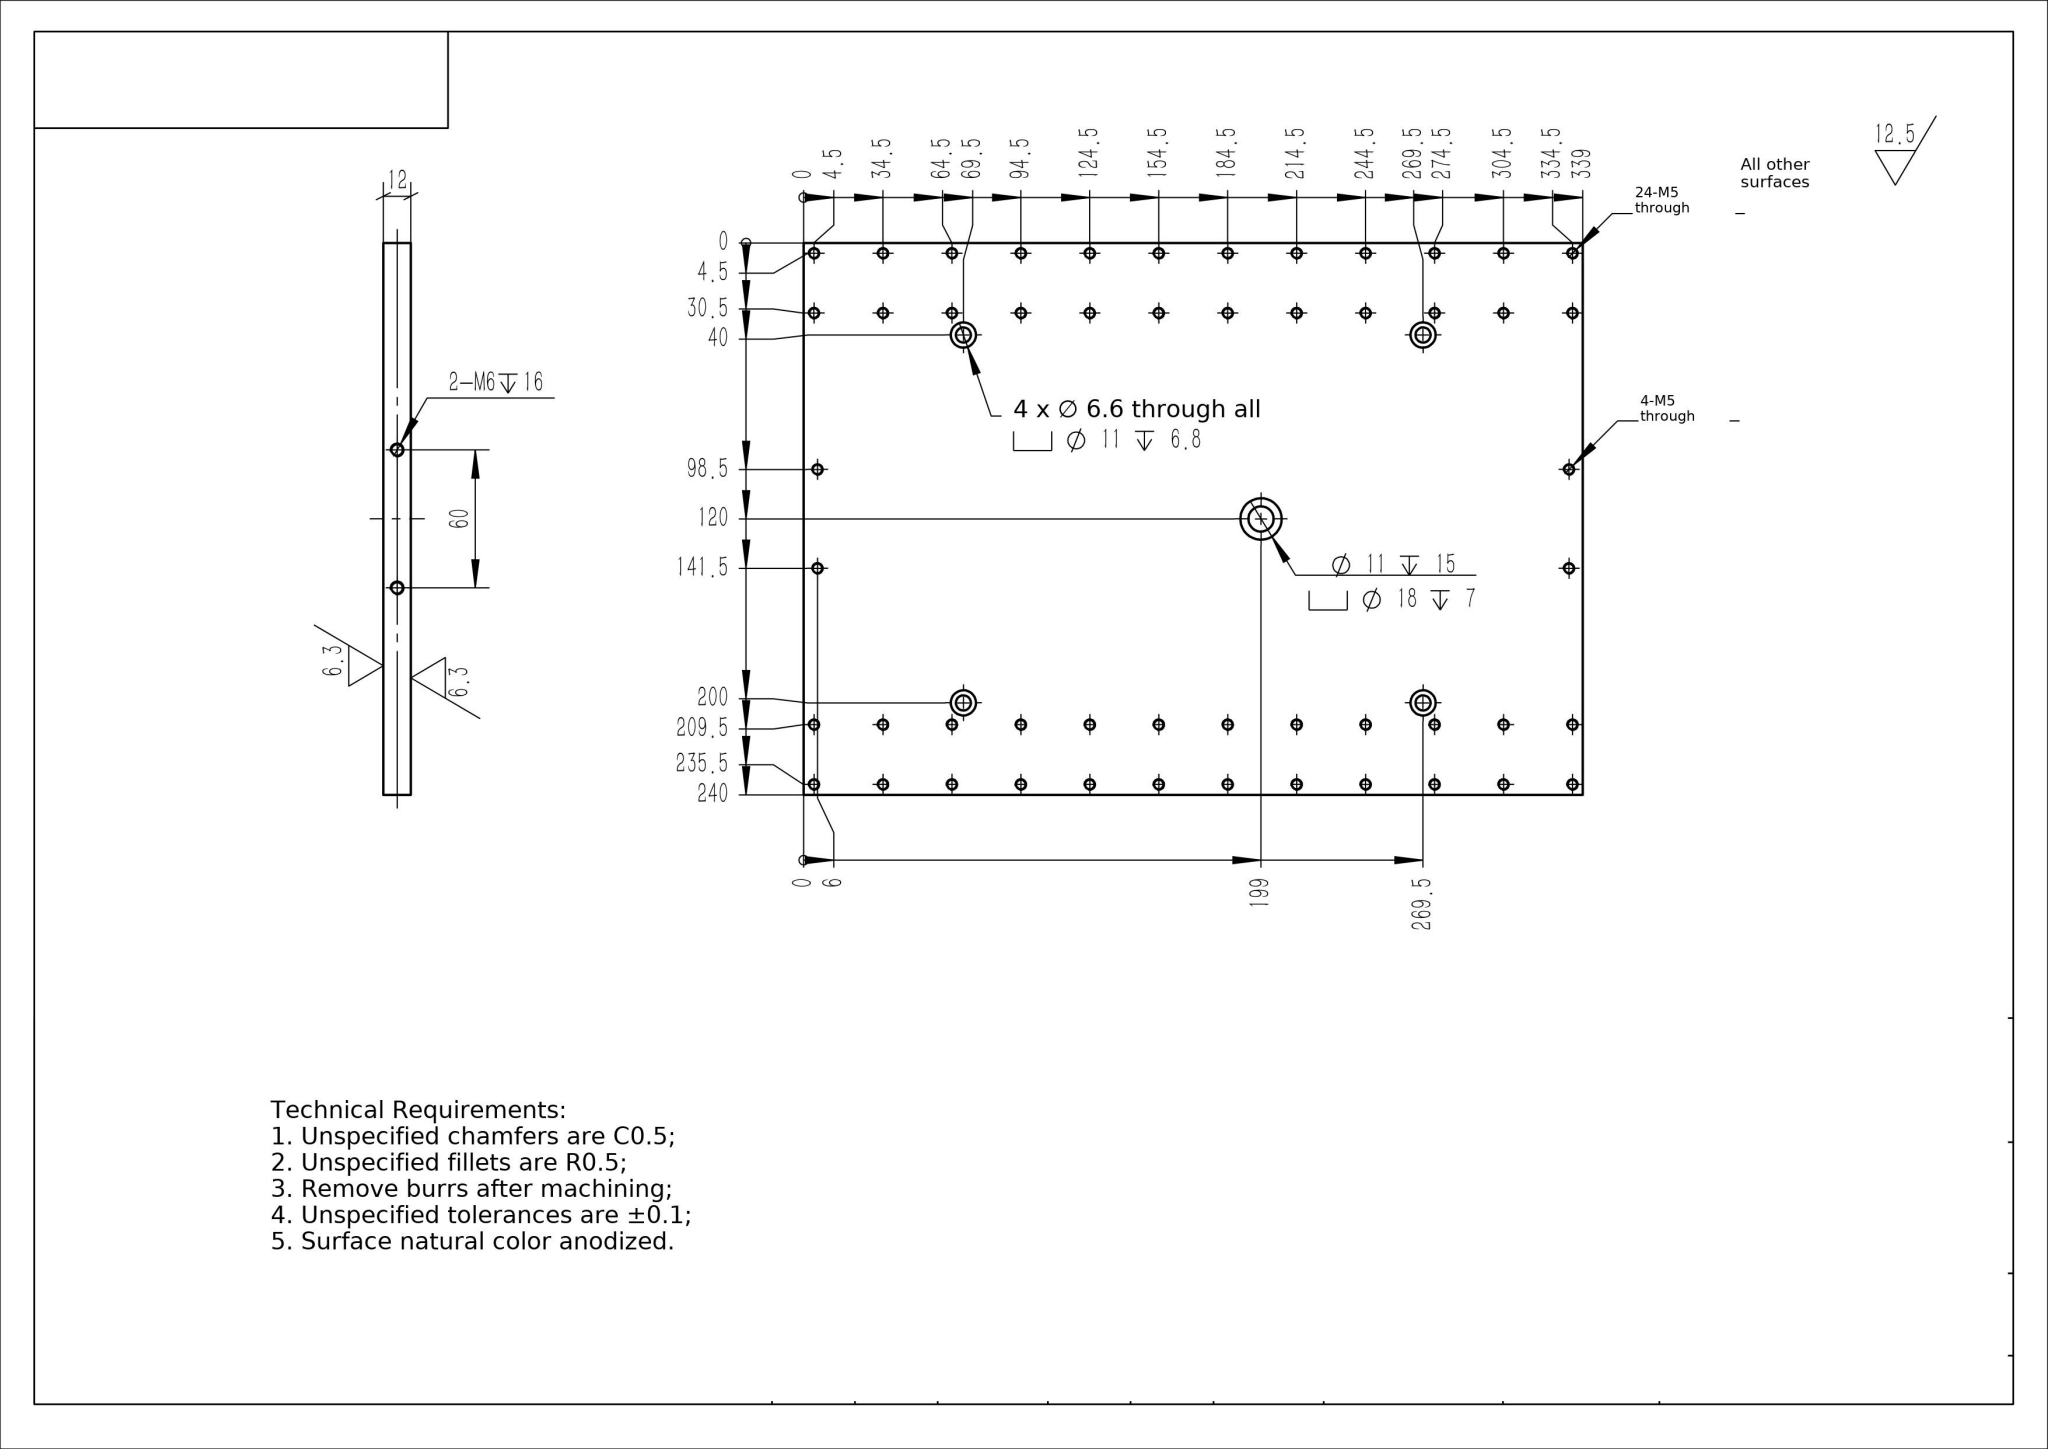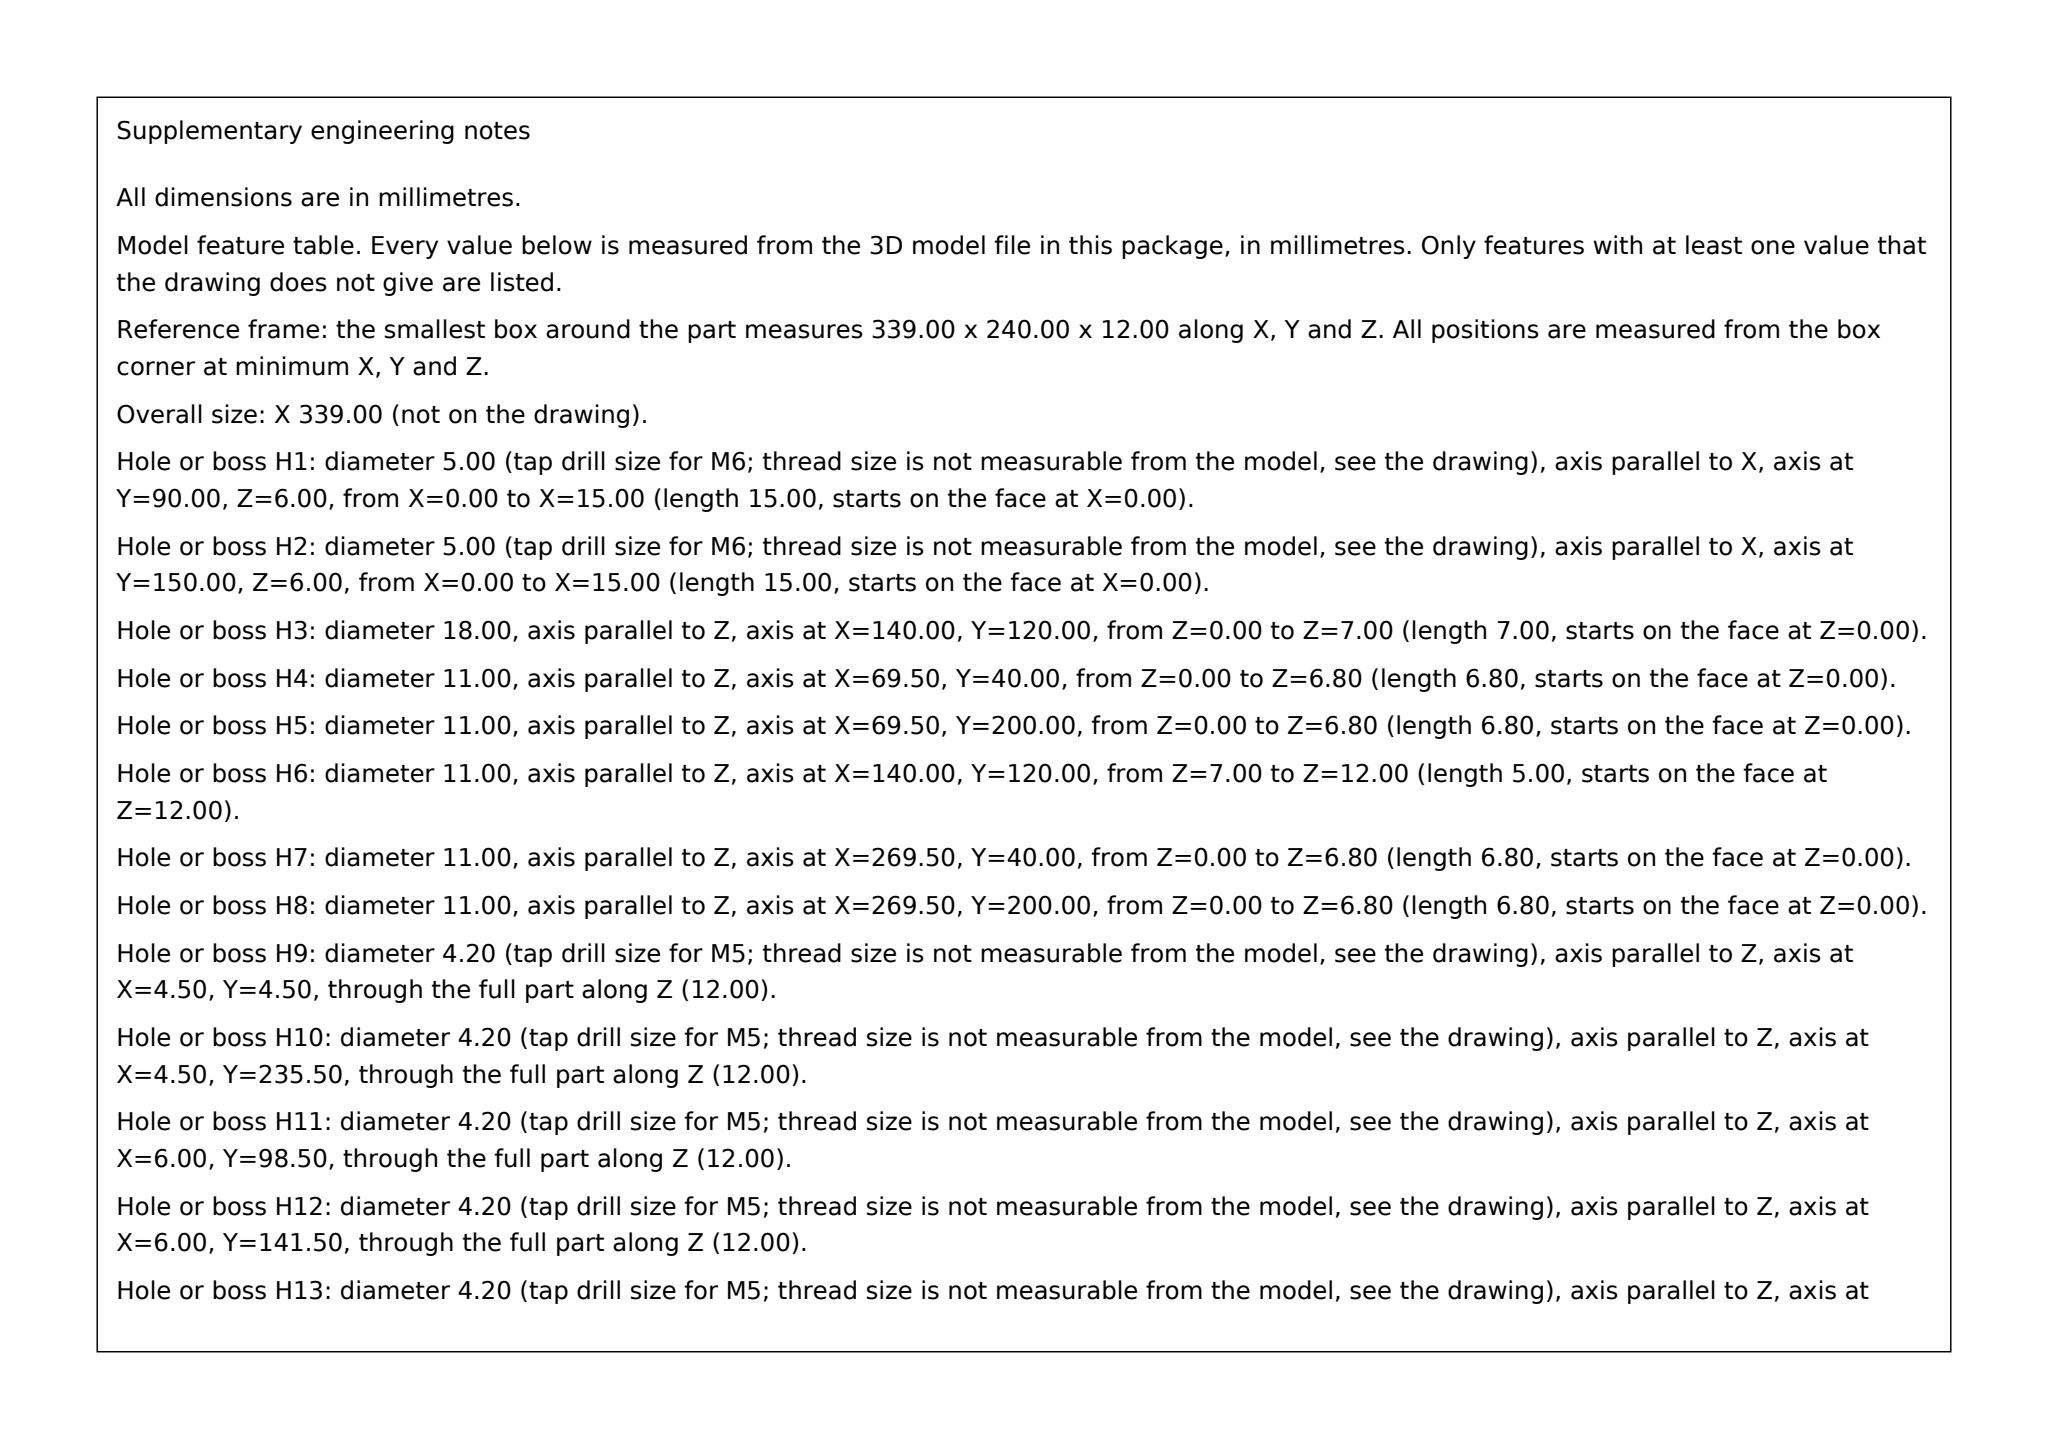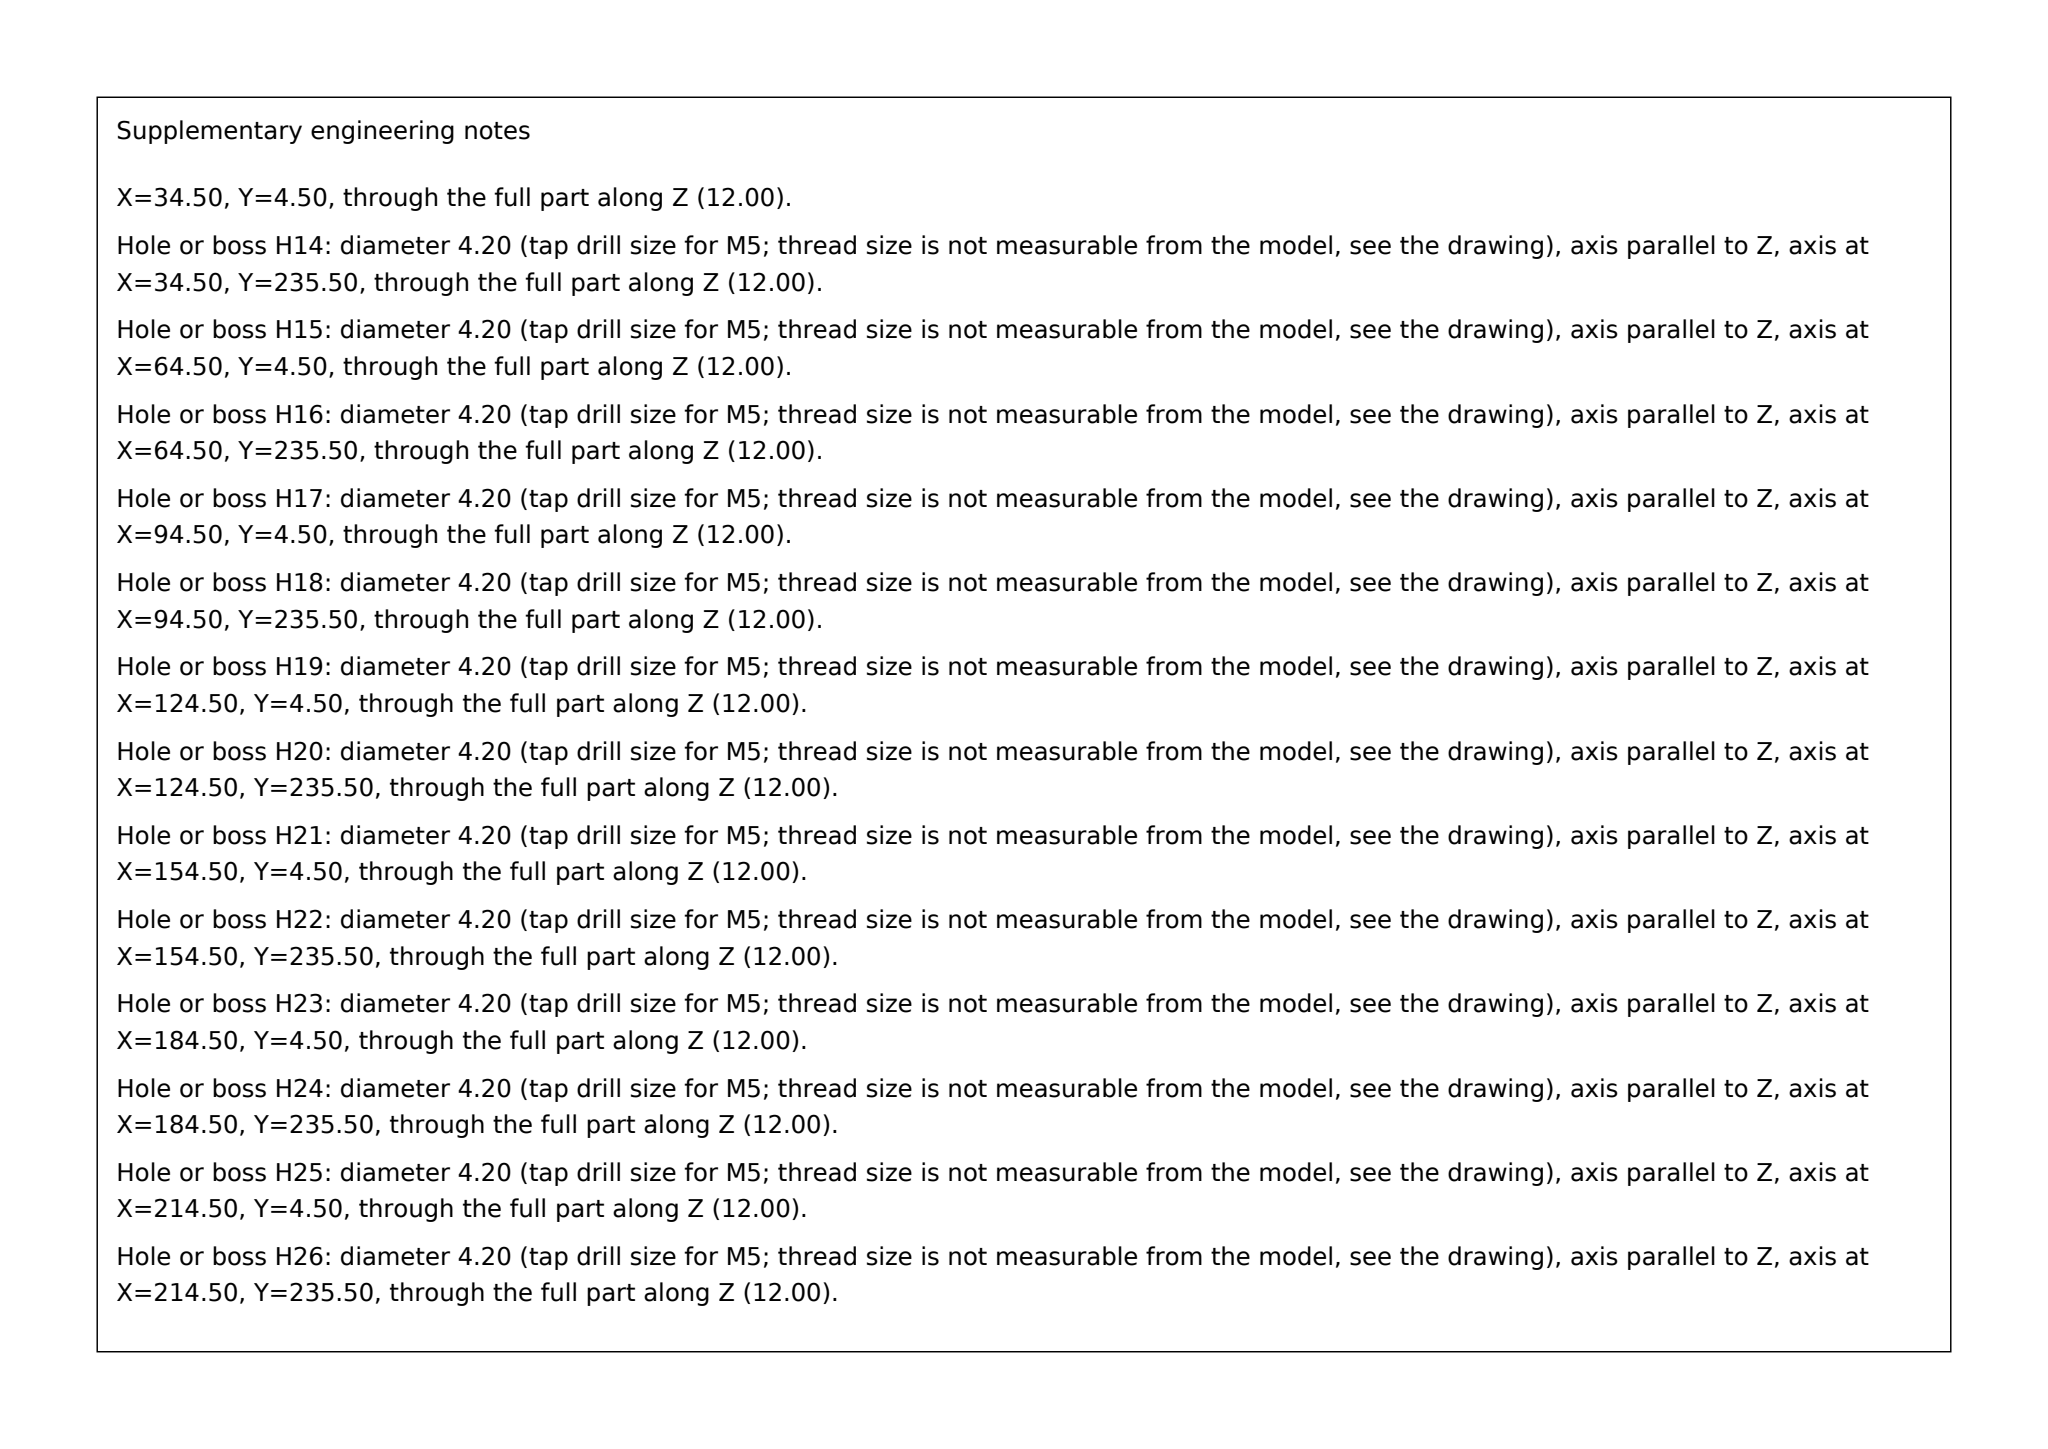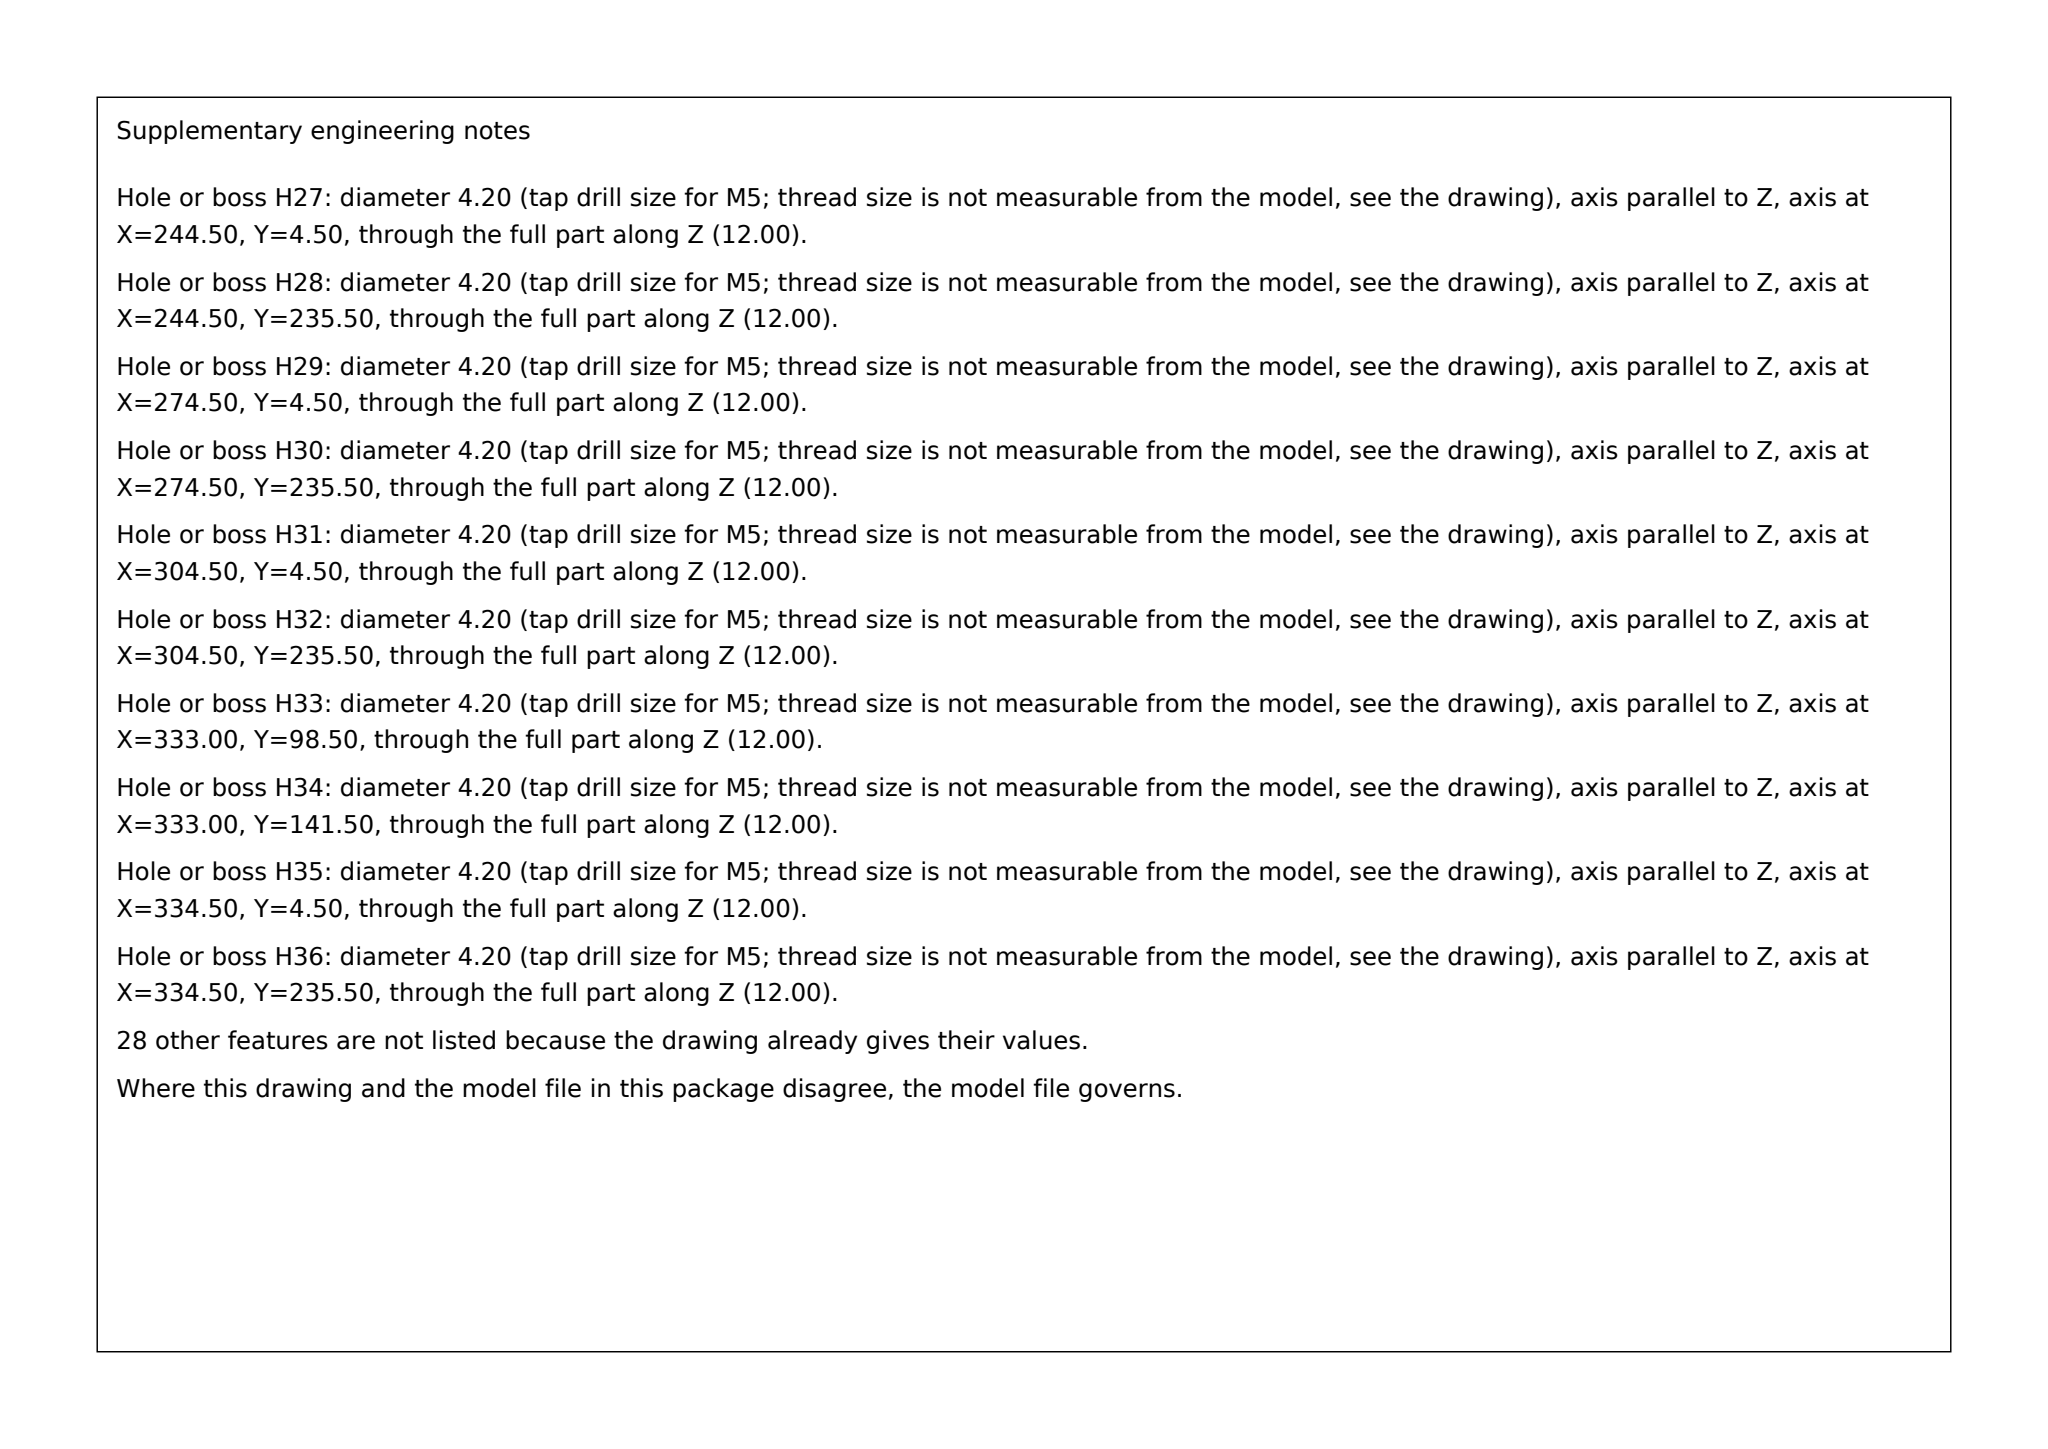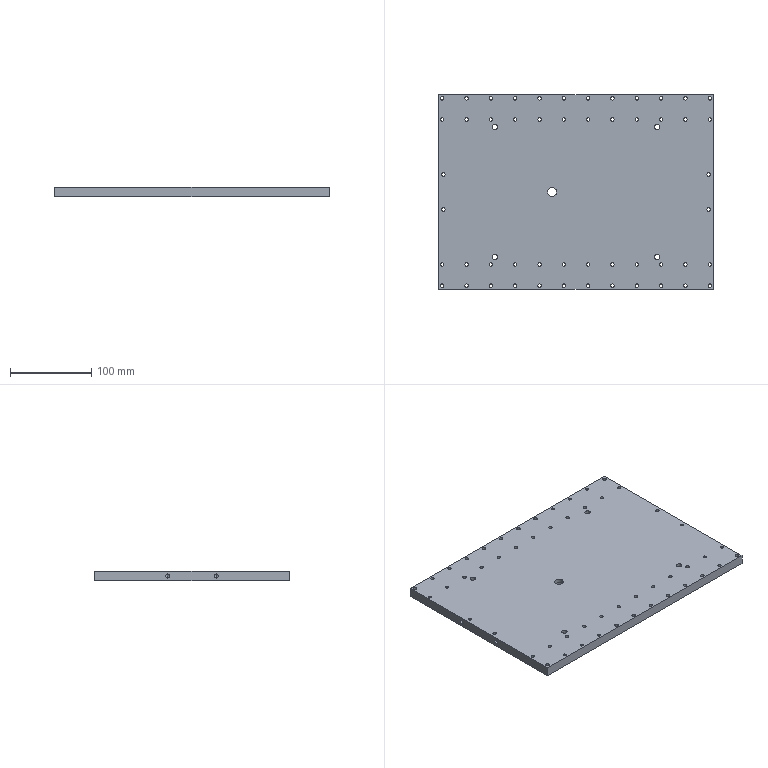Part | SolidWorks | mm | 1 solid | 143 faces | box 339 x 240 x 12 mm | volume 961513 mm3 | cylinder 128 | plane 11 | cone 4 | commonest cylinder face diameters 4.2 x104 11 x10 6.6 x8 5 x4 18 x2
build123d program:
from build123d import *

# Parameters (mm, degrees)
SKETCH1_W                                         = 339
SKETCH1_H                                         = 240
BOSS_EXTRUDE1_DEPTH                               = 12
M5_TAPPED_HOLE1_D                                 = 4.2
LPATTERN1_COUNT                                   = 6
LPATTERN1_PITCH                                   = 60
MIRROR1_COPY_1_D                                  = 4.2
MIRROR1_COPY_2_D                                  = 4.2
MIRROR1_COPY_3_D                                  = 4.2
MIRROR1_COPY_4_D                                  = 4.2
MIRROR1_COPY_5_D                                  = 4.2
M5_TAPPED_HOLE2_D                                 = 4.2
HOLE_SIZE_ACCORDING_TO_HEXAGON_SOCKET_D           = 6.6
HOLE_SIZE_ACCORDING_TO_HEXAGON_SOCKET_CBORE_D     = 11
HOLE_SIZE_ACCORDING_TO_HEXAGON_SOCKET_CBORE_DEPTH = 6.8
HOLE_SIZE_ACCORDING_TO_HEXAGON_SO_2_D             = 11
HOLE_SIZE_ACCORDING_TO_HEXAGON_SO_2_DEPTH         = 15
HOLE_SIZE_ACCORDING_TO_HEXAGON_SO_2_CBORE_D       = 18
HOLE_SIZE_ACCORDING_TO_HEXAGON_SO_2_CBORE_DEPTH   = 7
HOLE_SIZE_ACCORDING_TO_HEXAGON_SO_2_TIP           = 3.305
M6_TAPPED_HOLE1_D                                 = 5
M6_TAPPED_HOLE1_DEPTH                             = 15
M6_TAPPED_HOLE1_TIP                               = 1.502


with BuildPart() as part:
    # Sketch1 → Boss-Extrude1 (new body)
    with BuildSketch(Plane.XY):
        Rectangle(SKETCH1_W, SKETCH1_H)
    extrude(amount=BOSS_EXTRUDE1_DEPTH)

    # M5 Tapped Hole1 (through all)
    with Locations(Plane(origin=(0, 0, 0), x_dir=(1, 0, 0), z_dir=(0, 0, -1))):
        with Locations((-165, 115.5), (-165, 89.5), (-135, 89.5), (-135, 115.5)):
            m5_tapped_hole1 = Hole(M5_TAPPED_HOLE1_D / 2)

    # LPattern1: M5 Tapped Hole1 ×6
    with Locations(*[(i * LPATTERN1_PITCH, 0, 0) for i in range(1, LPATTERN1_COUNT)]):
        add(m5_tapped_hole1, mode=Mode.SUBTRACT)

    # Mirror1: M5 Tapped Hole1 across plane
    add(m5_tapped_hole1.mirror(Plane.ZX), mode=Mode.SUBTRACT)

    # Mirror1 copy 1 (through all)
    with Locations(Plane(origin=(60, 0, 0), x_dir=(1, 0, 0), z_dir=(0, 0, -1))):
        with Locations((-165, -115.5), (-165, -89.5), (-135, -89.5), (-135, -115.5)):
            Hole(MIRROR1_COPY_1_D / 2)

    # Mirror1 copy 2 (through all)
    with Locations(Plane(origin=(120, 0, 0), x_dir=(1, 0, 0), z_dir=(0, 0, -1))):
        with Locations((-165, -115.5), (-165, -89.5), (-135, -89.5), (-135, -115.5)):
            Hole(MIRROR1_COPY_2_D / 2)

    # Mirror1 copy 3 (through all)
    with Locations(Plane(origin=(180, 0, 0), x_dir=(1, 0, 0), z_dir=(0, 0, -1))):
        with Locations((-165, -115.5), (-165, -89.5), (-135, -89.5), (-135, -115.5)):
            Hole(MIRROR1_COPY_3_D / 2)

    # Mirror1 copy 4 (through all)
    with Locations(Plane(origin=(240, 0, 0), x_dir=(1, 0, 0), z_dir=(0, 0, -1))):
        with Locations((-165, -115.5), (-165, -89.5), (-135, -89.5), (-135, -115.5)):
            Hole(MIRROR1_COPY_4_D / 2)

    # Mirror1 copy 5 (through all)
    with Locations(Plane(origin=(300, 0, 0), x_dir=(1, 0, 0), z_dir=(0, 0, -1))):
        with Locations((-165, -115.5), (-165, -89.5), (-135, -89.5), (-135, -115.5)):
            Hole(MIRROR1_COPY_5_D / 2)

    # M5 Tapped Hole2 (through all)
    with Locations(Plane.XY.offset(12)):
        with Locations((-163.5, 21.5), (-163.5, -21.5), (163.5, -21.5), (163.5, 21.5)):
            Hole(M5_TAPPED_HOLE2_D / 2)

    # Hole Size _ according to_ Hexagon Socket (through all)
    with Locations(Plane(origin=(0, 0, 0), x_dir=(1, 0, 0), z_dir=(0, 0, -1))):
        with Locations((-100, -80), (100, -80), (100, 80), (-100, 80)):
            CounterBoreHole(HOLE_SIZE_ACCORDING_TO_HEXAGON_SOCKET_D / 2, HOLE_SIZE_ACCORDING_TO_HEXAGON_SOCKET_CBORE_D / 2, HOLE_SIZE_ACCORDING_TO_HEXAGON_SOCKET_CBORE_DEPTH)

    # Hole Size _ according to_ Hexagon So 2
    with Locations(Plane(origin=(0, 0, 0), x_dir=(-1, 0, 0), z_dir=(0, 0, -1))):
        with Locations((29.5, 0)):
            CounterBoreHole(HOLE_SIZE_ACCORDING_TO_HEXAGON_SO_2_D / 2, HOLE_SIZE_ACCORDING_TO_HEXAGON_SO_2_CBORE_D / 2, HOLE_SIZE_ACCORDING_TO_HEXAGON_SO_2_CBORE_DEPTH, depth=HOLE_SIZE_ACCORDING_TO_HEXAGON_SO_2_DEPTH)
            with Locations((0, 0, -(HOLE_SIZE_ACCORDING_TO_HEXAGON_SO_2_DEPTH + HOLE_SIZE_ACCORDING_TO_HEXAGON_SO_2_TIP / 2))):  # 118° drill point
                Cone(0, HOLE_SIZE_ACCORDING_TO_HEXAGON_SO_2_D / 2, HOLE_SIZE_ACCORDING_TO_HEXAGON_SO_2_TIP, mode=Mode.SUBTRACT)

    # M6 Tapped Hole1
    with Locations(Plane.ZY.offset(169.5)):
        with Locations((6, -30), (6, 30)):
            Hole(M6_TAPPED_HOLE1_D / 2, depth=M6_TAPPED_HOLE1_DEPTH)
            with Locations((0, 0, -(M6_TAPPED_HOLE1_DEPTH + M6_TAPPED_HOLE1_TIP / 2))):  # 118° drill point
                Cone(0, M6_TAPPED_HOLE1_D / 2, M6_TAPPED_HOLE1_TIP, mode=Mode.SUBTRACT)


solid = part.part